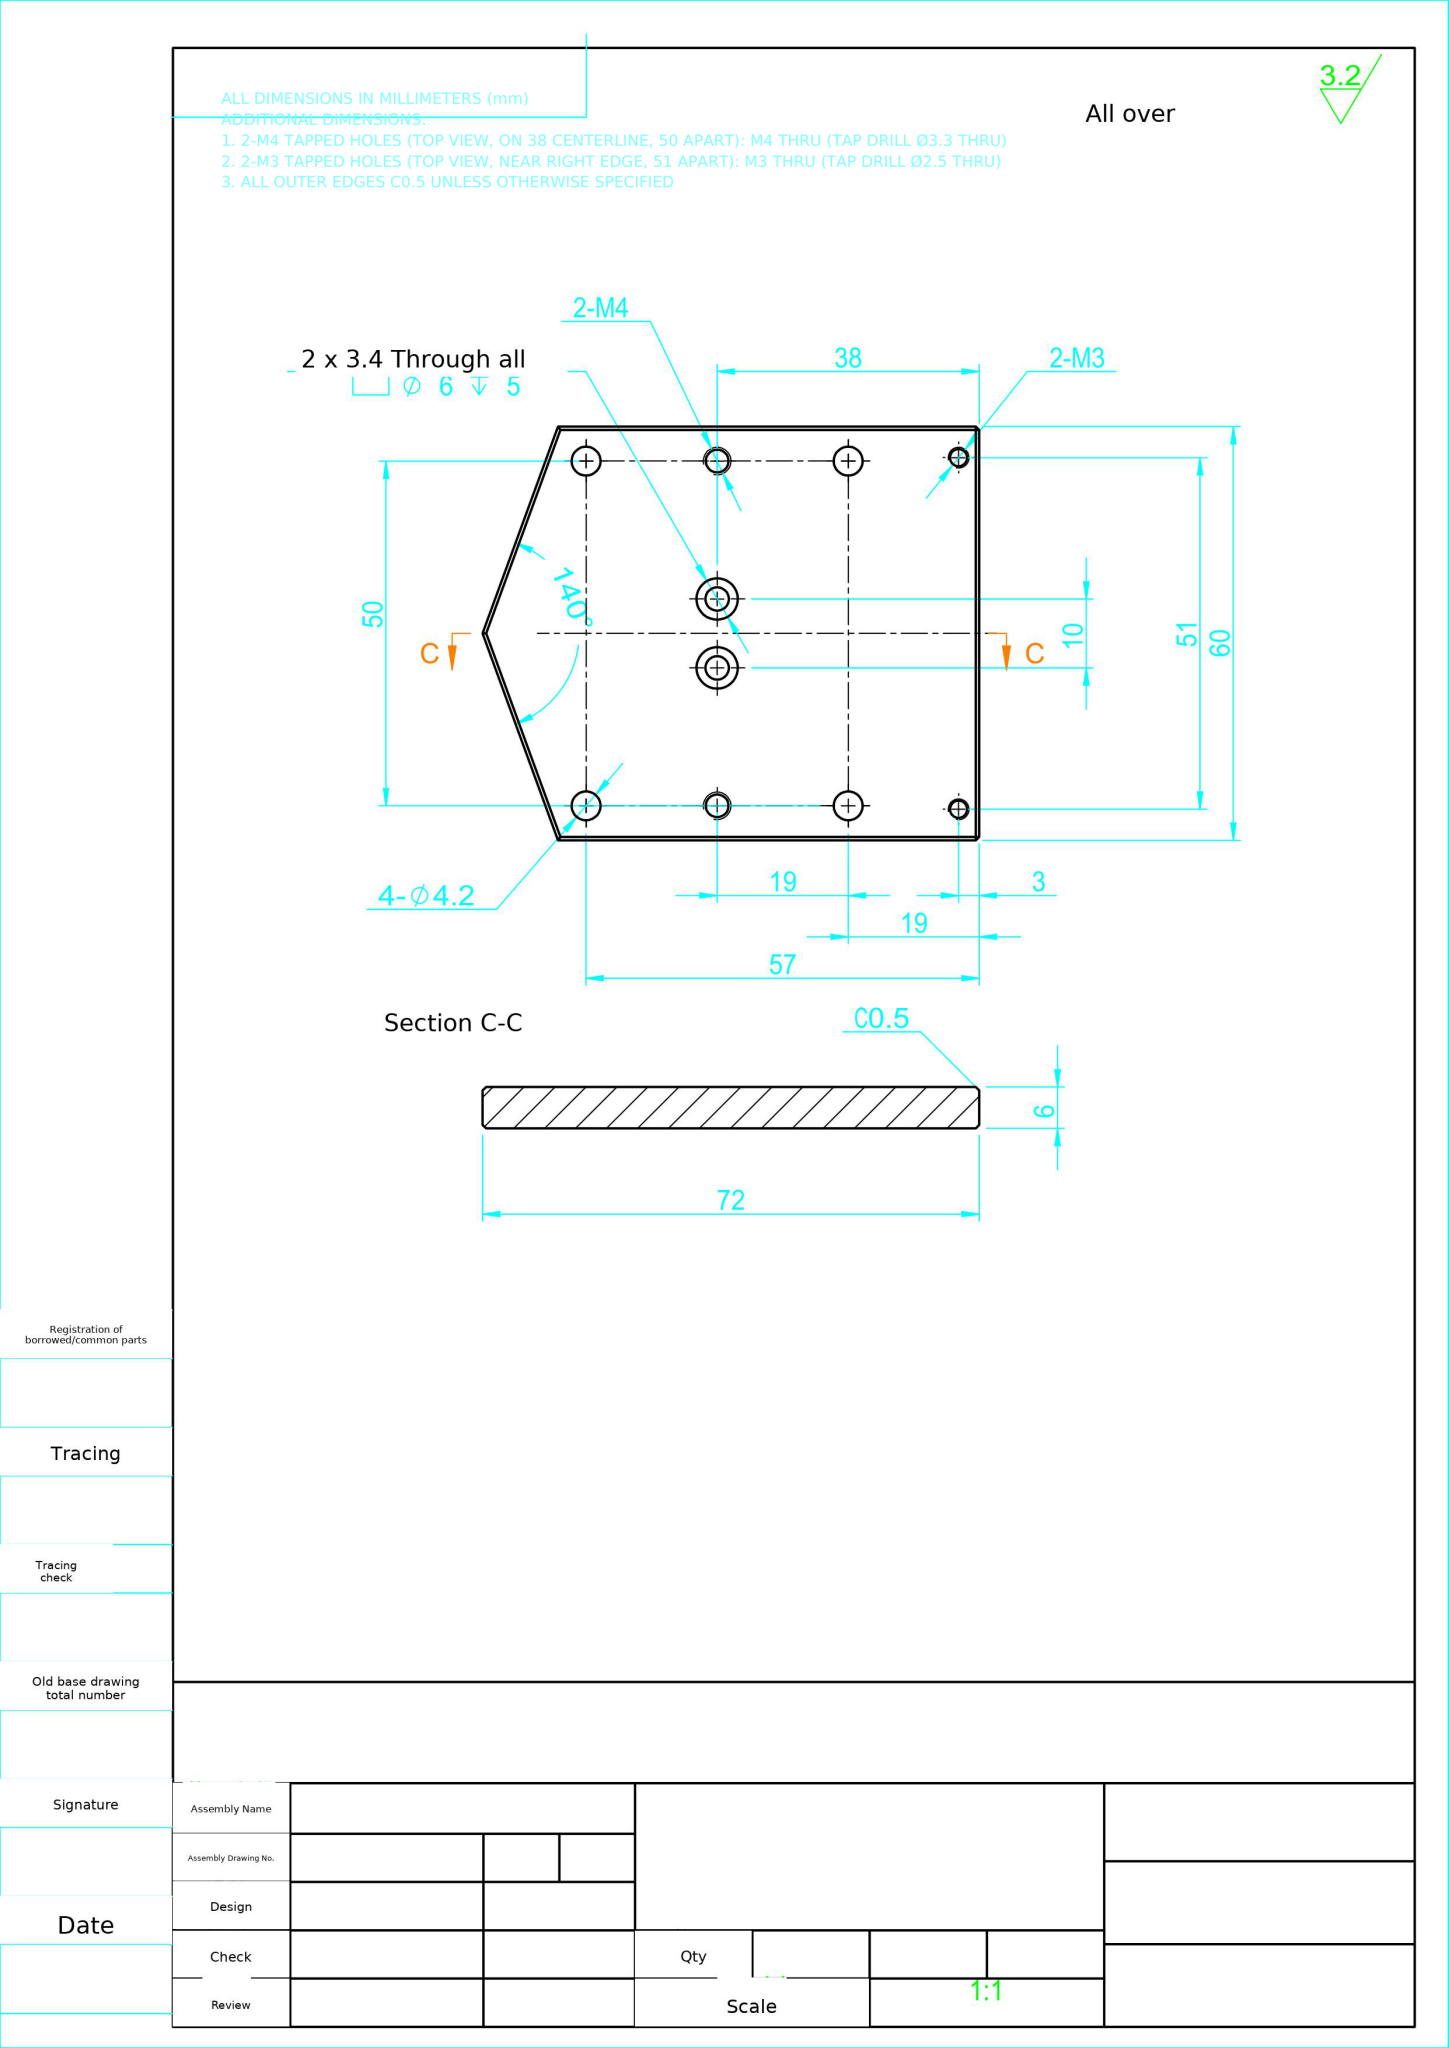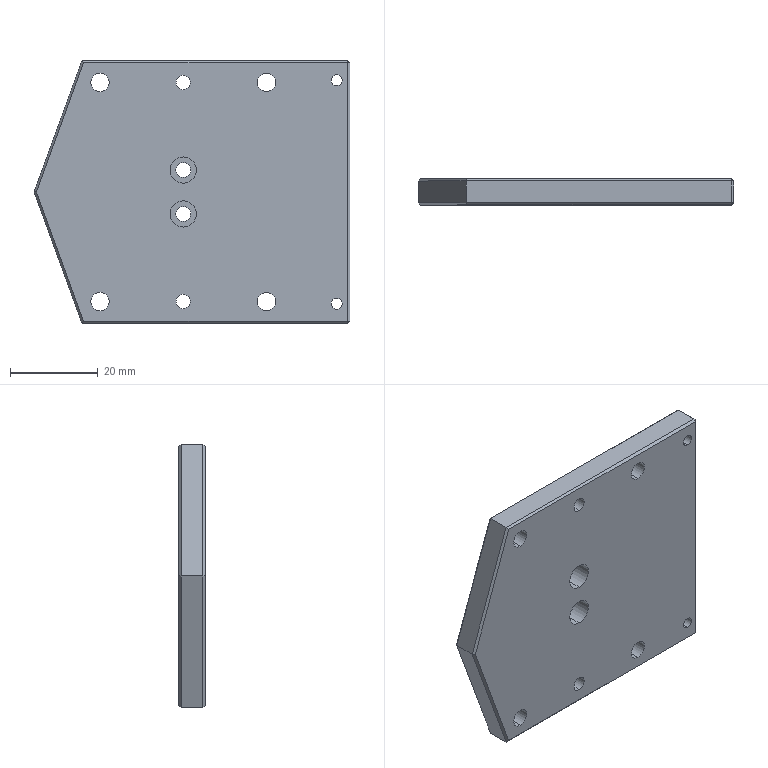Part | NX | mm | 1 solid | 49 faces | box 72 x 6 x 60 mm | volume 23097 mm3 | plane 25 | cylinder 24 | commonest cylinder face diameters 4.2 x8 2.5 x4 3.3 x4 6 x4 3.4 x4